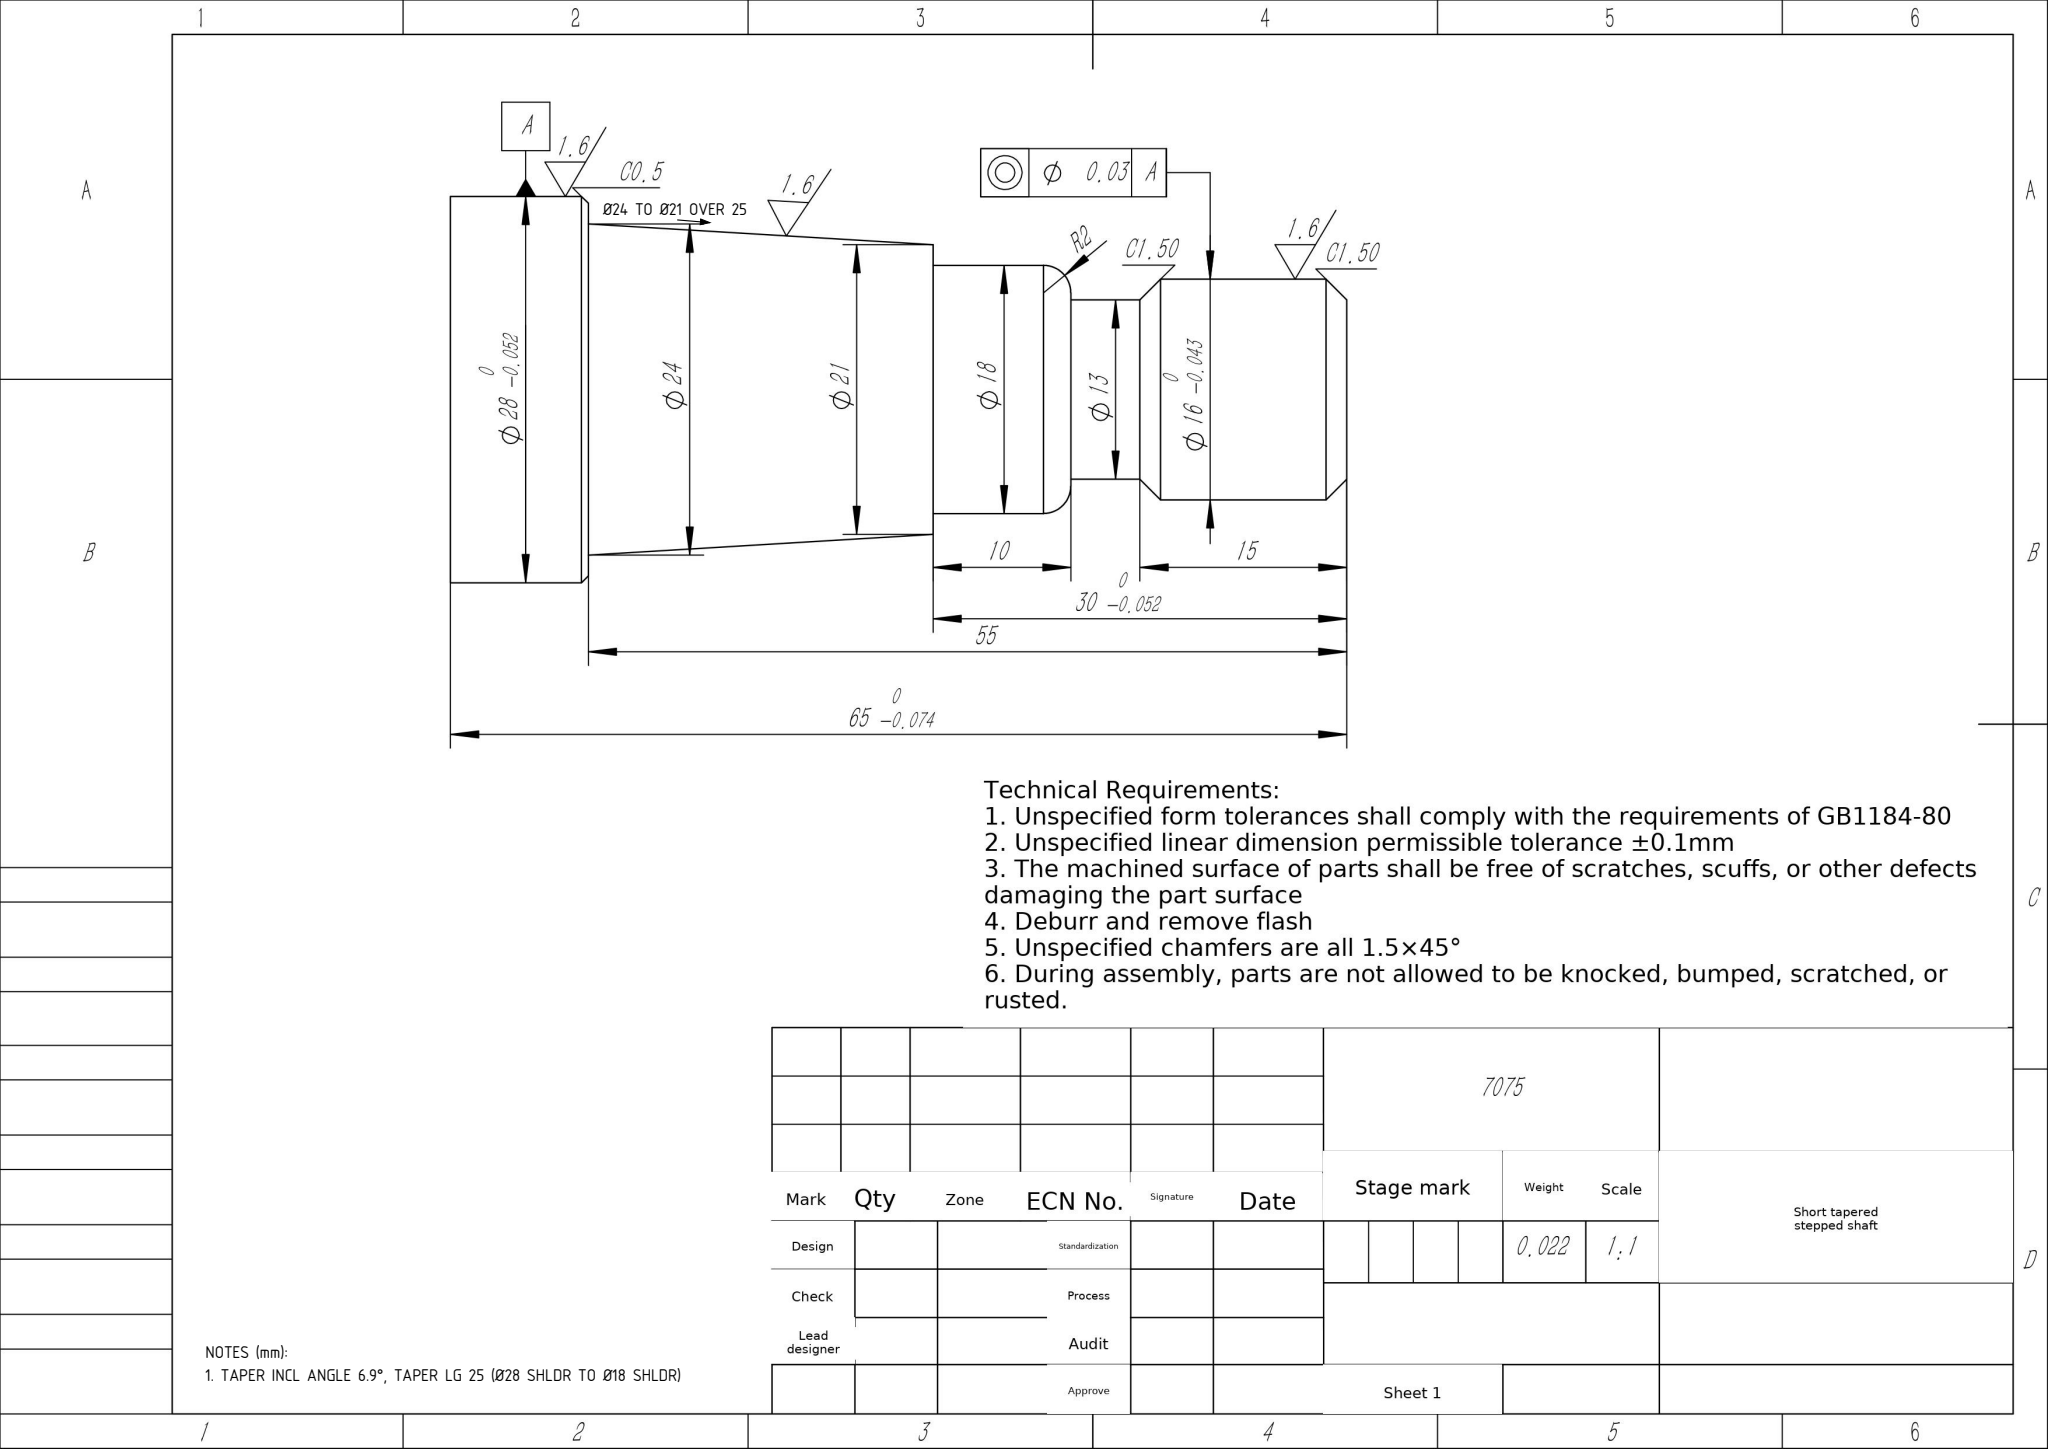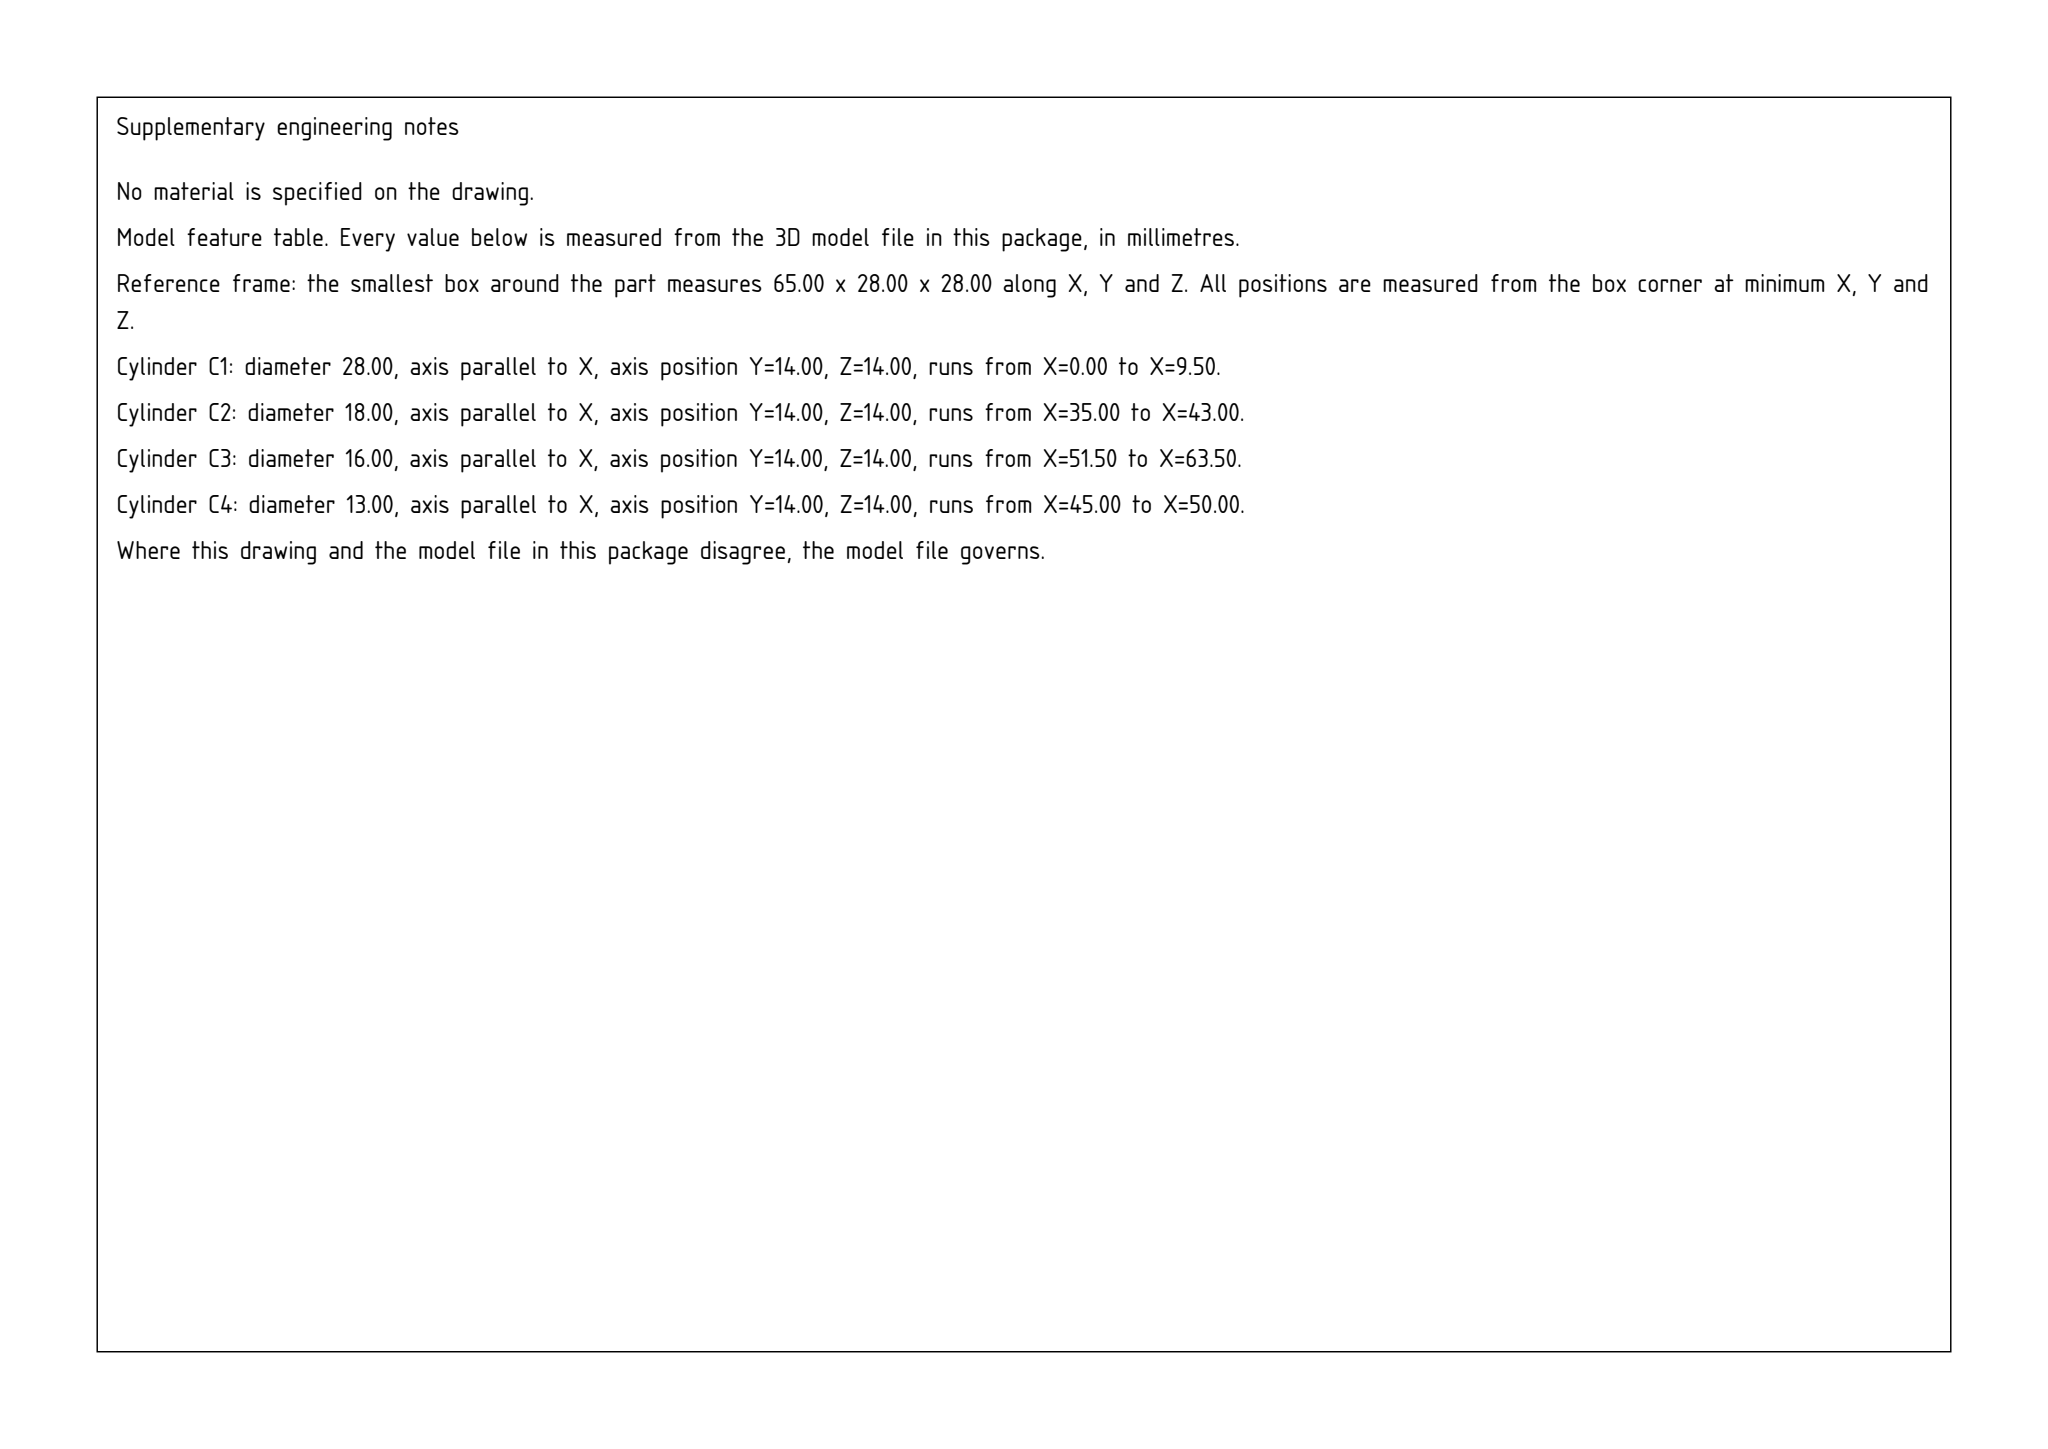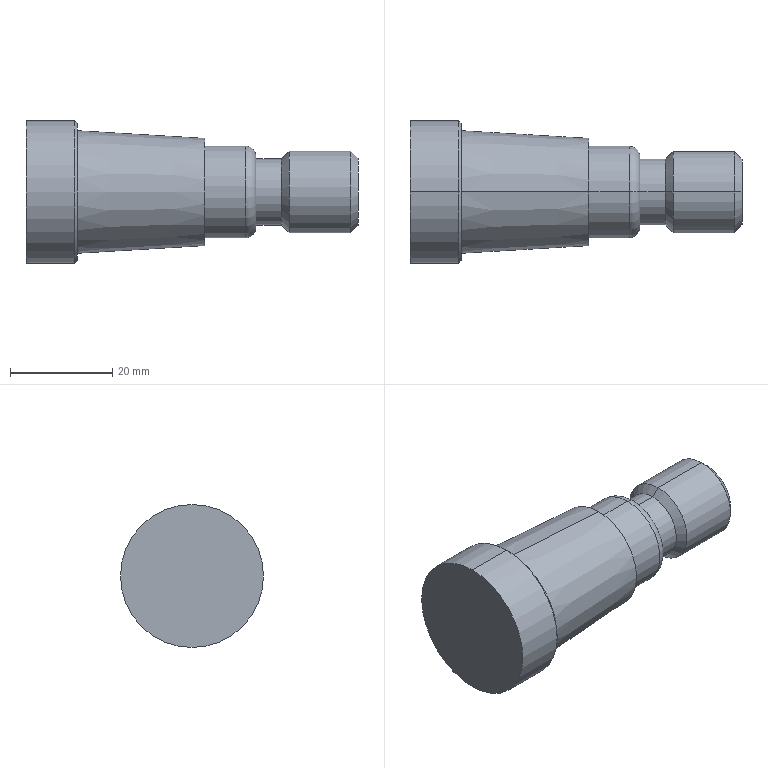Part | SolidWorks | mm | material 7075 | 1 solid | 23 faces | box 65 x 28 x 28 mm | volume 22174 mm3 | cone 8 | cylinder 8 | plane 5 | torus 2 | commonest cylinder face diameters 16 x2 13 x2 18 x2 28 x2
Drawing notes:
TAPER: Ø24 AT Ø28 SHLDR FACE, Ø21 AT 25 FROM THAT FACE | from the solid: Cone ref dia 21, spans planes x=10 to x=35; Ø28 cyl ends x=9.5/face x=10; dia change 3 over 25
TAPER INCL ANGLE 6.9°, TAPER LG 25 (Ø28 SHLDR TO Ø18 SHLDR) | from the solid: cones[included_angle,ref_dia]=[6.9,21]; axis planes x=10 and x=35 -> 25 long
STEP:
#1=CARTESIAN_POINT('',(10.,0.,-13.5));
#2=VERTEX_POINT('',#1);
#3=CARTESIAN_POINT('',(10.,0.,13.5));
#4=VERTEX_POINT('',#3);
#5=CARTESIAN_POINT('',(10.,0.,0.));
#6=DIRECTION('',(1.,0.,0.));
#7=DIRECTION('',(0.,0.,1.));
#8=AXIS2_PLACEMENT_3D('',#5,#6,#7);
#9=CIRCLE('',#8,13.5);
#10=EDGE_CURVE('',#2,#4,#9,.T.);
#11=ORIENTED_EDGE('',*,*,#10,.F.);
#12=CARTESIAN_POINT('',(9.5,0.,-14.));
#13=VERTEX_POINT('',#12);
#14=CARTESIAN_POINT('',(9.5,0.,-14.));
#15=DIRECTION('',(-0.7071,0.,-0.7071));
#16=VECTOR('',#15,1000.);
#17=LINE('',#14,#16);
#18=EDGE_CURVE('',#2,#13,#17,.T.);
#19=ORIENTED_EDGE('',*,*,#18,.T.);
#20=CARTESIAN_POINT('',(9.5,0.,14.));
#21=VERTEX_POINT('',#20);
#22=CARTESIAN_POINT('',(9.5,0.,0.));
#23=DIRECTION('',(-1.,0.,0.));
#24=DIRECTION('',(0.,0.,1.));
#25=AXIS2_PLACEMENT_3D('',#22,#23,#24);
#26=CIRCLE('',#25,14.);
#27=EDGE_CURVE('',#21,#13,#26,.T.);
#28=ORIENTED_EDGE('',*,*,#27,.F.);
#29=CARTESIAN_POINT('',(9.5,0.,14.));
#30=DIRECTION('',(-0.7071,0.,0.7071));
#31=VECTOR('',#30,1000.);
#32=LINE('',#29,#31);
#33=EDGE_CURVE('',#4,#21,#32,.T.);
#34=ORIENTED_EDGE('',*,*,#33,.F.);
#35=EDGE_LOOP('',(#11,#19,#28,#34));
#36=FACE_OUTER_BOUND('',#35,.T.);
#37=CARTESIAN_POINT('',(9.5,0.,0.));
#38=DIRECTION('',(-1.,0.,0.));
#39=DIRECTION('',(0.,0.,1.));
#40=AXIS2_PLACEMENT_3D('',#37,#38,#39);
#41=CONICAL_SURFACE('',#40,14.,0.7854);
#42=ADVANCED_FACE('',(#36),#41,.T.);
#43=CARTESIAN_POINT('',(45.,0.,-7.));
#44=VERTEX_POINT('',#43);
#45=CARTESIAN_POINT('',(45.,0.,7.));
#46=VERTEX_POINT('',#45);
#47=CARTESIAN_POINT('',(45.,0.,0.));
#48=DIRECTION('',(1.,0.,0.));
#49=DIRECTION('',(0.,0.,1.));
#50=AXIS2_PLACEMENT_3D('',#47,#48,#49);
#51=CIRCLE('',#50,7.);
#52=EDGE_CURVE('',#44,#46,#51,.T.);
#53=ORIENTED_EDGE('',*,*,#52,.F.);
#54=CARTESIAN_POINT('',(43.,0.,-9.));
#55=VERTEX_POINT('',#54);
#56=CARTESIAN_POINT('',(43.,0.,-7.));
#57=DIRECTION('',(0.,1.,0.));
#58=DIRECTION('',(0.,-0.,1.));
#59=AXIS2_PLACEMENT_3D('',#56,#57,#58);
#60=CIRCLE('',#59,2.);
#61=EDGE_CURVE('',#44,#55,#60,.T.);
#62=ORIENTED_EDGE('',*,*,#61,.T.);
#63=CARTESIAN_POINT('',(43.,0.,9.));
#64=VERTEX_POINT('',#63);
#65=CARTESIAN_POINT('',(43.,0.,0.));
#66=DIRECTION('',(-1.,0.,0.));
#67=DIRECTION('',(0.,0.,1.));
#68=AXIS2_PLACEMENT_3D('',#65,#66,#67);
#69=CIRCLE('',#68,9.);
#70=EDGE_CURVE('',#64,#55,#69,.T.);
#71=ORIENTED_EDGE('',*,*,#70,.F.);
#72=CARTESIAN_POINT('',(43.,0.,7.));
#73=DIRECTION('',(0.,-1.,0.));
#74=DIRECTION('',(0.,0.,-1.));
#75=AXIS2_PLACEMENT_3D('',#72,#73,#74);
#76=CIRCLE('',#75,2.);
#77=EDGE_CURVE('',#46,#64,#76,.T.);
#78=ORIENTED_EDGE('',*,*,#77,.F.);
#79=EDGE_LOOP('',(#53,#62,#71,#78));
#80=FACE_OUTER_BOUND('',#79,.T.);
#81=CARTESIAN_POINT('',(43.,0.,0.));
#82=DIRECTION('',(-1.,0.,0.));
#83=DIRECTION('',(0.,0.,1.));
#84=AXIS2_PLACEMENT_3D('',#81,#82,#83);
#85=TOROIDAL_SURFACE('',#84,7.,2.);
#86=ADVANCED_FACE('',(#80),#85,.T.);
#87=CARTESIAN_POINT('',(50.,0.,6.5));
#88=VERTEX_POINT('',#87);
#89=CARTESIAN_POINT('',(50.,0.,-6.5));
#90=VERTEX_POINT('',#89);
#91=CARTESIAN_POINT('',(50.,0.,0.));
#92=DIRECTION('',(-1.,0.,0.));
#93=DIRECTION('',(0.,0.,1.));
#94=AXIS2_PLACEMENT_3D('',#91,#92,#93);
#95=CIRCLE('',#94,6.5);
#96=EDGE_CURVE('',#88,#90,#95,.T.);
#97=ORIENTED_EDGE('',*,*,#96,.F.);
#98=CARTESIAN_POINT('',(51.5,0.,8.));
#99=VERTEX_POINT('',#98);
#100=CARTESIAN_POINT('',(50.,0.,6.5));
#101=DIRECTION('',(0.7071,0.,0.7071));
#102=VECTOR('',#101,1000.);
#103=LINE('',#100,#102);
#104=EDGE_CURVE('',#88,#99,#103,.T.);
#105=ORIENTED_EDGE('',*,*,#104,.T.);
#106=CARTESIAN_POINT('',(51.5,0.,-8.));
#107=VERTEX_POINT('',#106);
#108=CARTESIAN_POINT('',(51.5,0.,0.));
#109=DIRECTION('',(1.,0.,0.));
#110=DIRECTION('',(0.,0.,-1.));
#111=AXIS2_PLACEMENT_3D('',#108,#109,#110);
#112=CIRCLE('',#111,8.);
#113=EDGE_CURVE('',#107,#99,#112,.T.);
#114=ORIENTED_EDGE('',*,*,#113,.F.);
#115=CARTESIAN_POINT('',(50.,0.,-6.5));
#116=DIRECTION('',(0.7071,0.,-0.7071));
#117=VECTOR('',#116,1000.);
#118=LINE('',#115,#117);
#119=EDGE_CURVE('',#90,#107,#118,.T.);
#120=ORIENTED_EDGE('',*,*,#119,.F.);
#121=EDGE_LOOP('',(#97,#105,#114,#120));
#122=FACE_OUTER_BOUND('',#121,.T.);
#123=CARTESIAN_POINT('',(50.,0.,0.));
#124=DIRECTION('',(1.,0.,0.));
#125=DIRECTION('',(0.,0.,-1.));
#126=AXIS2_PLACEMENT_3D('',#123,#124,#125);
#127=CONICAL_SURFACE('',#126,6.5,0.7854);
#128=ADVANCED_FACE('',(#122),#127,.T.);
#129=CARTESIAN_POINT('',(65.,0.,-6.5));
#130=VERTEX_POINT('',#129);
#131=CARTESIAN_POINT('',(65.,0.,6.5));
#132=VERTEX_POINT('',#131);
#133=CARTESIAN_POINT('',(65.,0.,0.));
#134=DIRECTION('',(1.,0.,0.));
#135=DIRECTION('',(0.,0.,1.));
#136=AXIS2_PLACEMENT_3D('',#133,#134,#135);
#137=CIRCLE('',#136,6.5);
#138=EDGE_CURVE('',#130,#132,#137,.T.);
#139=ORIENTED_EDGE('',*,*,#138,.F.);
#140=CARTESIAN_POINT('',(63.5,0.,-8.));
#141=VERTEX_POINT('',#140);
#142=CARTESIAN_POINT('',(63.5,0.,-8.));
#143=DIRECTION('',(-0.7071,0.,-0.7071));
#144=VECTOR('',#143,1000.);
#145=LINE('',#142,#144);
#146=EDGE_CURVE('',#130,#141,#145,.T.);
#147=ORIENTED_EDGE('',*,*,#146,.T.);
#148=CARTESIAN_POINT('',(63.5,0.,8.));
#149=VERTEX_POINT('',#148);
#150=CARTESIAN_POINT('',(63.5,0.,0.));
#151=DIRECTION('',(-1.,0.,0.));
#152=DIRECTION('',(0.,0.,1.));
#153=AXIS2_PLACEMENT_3D('',#150,#151,#152);
#154=CIRCLE('',#153,8.);
#155=EDGE_CURVE('',#149,#141,#154,.T.);
#156=ORIENTED_EDGE('',*,*,#155,.F.);
#157=CARTESIAN_POINT('',(63.5,0.,8.));
#158=DIRECTION('',(-0.7071,0.,0.7071));
#159=VECTOR('',#158,1000.);
#160=LINE('',#157,#159);
#161=EDGE_CURVE('',#132,#149,#160,.T.);
#162=ORIENTED_EDGE('',*,*,#161,.F.);
#163=EDGE_LOOP('',(#139,#147,#156,#162));
#164=FACE_OUTER_BOUND('',#163,.T.);
#165=CARTESIAN_POINT('',(63.5,0.,0.));
#166=DIRECTION('',(-1.,0.,0.));
#167=DIRECTION('',(0.,0.,1.));
#168=AXIS2_PLACEMENT_3D('',#165,#166,#167);
#169=CONICAL_SURFACE('',#168,8.,0.7854);
#170=ADVANCED_FACE('',(#164),#169,.T.);
#171=ORIENTED_EDGE('',*,*,#155,.T.);
#172=CARTESIAN_POINT('',(0.,0.,-8.));
#173=DIRECTION('',(-1.,0.,0.));
#174=VECTOR('',#173,1000.);
#175=LINE('',#172,#174);
#176=EDGE_CURVE('',#141,#107,#175,.T.);
#177=ORIENTED_EDGE('',*,*,#176,.T.);
#178=ORIENTED_EDGE('',*,*,#113,.T.);
#179=CARTESIAN_POINT('',(0.,0.,8.));
#180=DIRECTION('',(-1.,0.,0.));
#181=VECTOR('',#180,1000.);
#182=LINE('',#179,#181);
#183=EDGE_CURVE('',#149,#99,#182,.T.);
#184=ORIENTED_EDGE('',*,*,#183,.F.);
#185=EDGE_LOOP('',(#171,#177,#178,#184));
#186=FACE_OUTER_BOUND('',#185,.T.);
#187=CARTESIAN_POINT('',(0.,0.,0.));
#188=DIRECTION('',(-1.,0.,0.));
#189=DIRECTION('',(0.,0.,1.));
#190=AXIS2_PLACEMENT_3D('',#187,#188,#189);
#191=CYLINDRICAL_SURFACE('',#190,8.);
#192=ADVANCED_FACE('',(#186),#191,.T.);
#193=ORIENTED_EDGE('',*,*,#96,.T.);
#194=CARTESIAN_POINT('',(45.,0.,-6.5));
#195=VERTEX_POINT('',#194);
#196=CARTESIAN_POINT('',(0.,0.,-6.5));
#197=DIRECTION('',(-1.,0.,0.));
#198=VECTOR('',#197,1000.);
#199=LINE('',#196,#198);
#200=EDGE_CURVE('',#90,#195,#199,.T.);
#201=ORIENTED_EDGE('',*,*,#200,.T.);
#202=CARTESIAN_POINT('',(45.,0.,6.5));
#203=VERTEX_POINT('',#202);
#204=CARTESIAN_POINT('',(45.,0.,0.));
#205=DIRECTION('',(-1.,0.,0.));
#206=DIRECTION('',(0.,0.,1.));
#207=AXIS2_PLACEMENT_3D('',#204,#205,#206);
#208=CIRCLE('',#207,6.5);
#209=EDGE_CURVE('',#203,#195,#208,.T.);
#210=ORIENTED_EDGE('',*,*,#209,.F.);
#211=CARTESIAN_POINT('',(0.,0.,6.5));
#212=DIRECTION('',(-1.,0.,0.));
#213=VECTOR('',#212,1000.);
#214=LINE('',#211,#213);
#215=EDGE_CURVE('',#88,#203,#214,.T.);
#216=ORIENTED_EDGE('',*,*,#215,.F.);
#217=EDGE_LOOP('',(#193,#201,#210,#216));
#218=FACE_OUTER_BOUND('',#217,.T.);
#219=CARTESIAN_POINT('',(0.,0.,0.));
#220=DIRECTION('',(-1.,0.,0.));
#221=DIRECTION('',(0.,0.,1.));
#222=AXIS2_PLACEMENT_3D('',#219,#220,#221);
#223=CYLINDRICAL_SURFACE('',#222,6.5);
#224=ADVANCED_FACE('',(#218),#223,.T.);
#225=ORIENTED_EDGE('',*,*,#70,.T.);
#226=CARTESIAN_POINT('',(35.,0.,-9.));
#227=VERTEX_POINT('',#226);
#228=CARTESIAN_POINT('',(0.,0.,-9.));
#229=DIRECTION('',(-1.,0.,0.));
#230=VECTOR('',#229,1000.);
#231=LINE('',#228,#230);
#232=EDGE_CURVE('',#55,#227,#231,.T.);
#233=ORIENTED_EDGE('',*,*,#232,.T.);
#234=CARTESIAN_POINT('',(35.,0.,9.));
#235=VERTEX_POINT('',#234);
#236=CARTESIAN_POINT('',(35.,0.,0.));
#237=DIRECTION('',(-1.,0.,0.));
#238=DIRECTION('',(0.,0.,1.));
#239=AXIS2_PLACEMENT_3D('',#236,#237,#238);
#240=CIRCLE('',#239,9.);
#241=EDGE_CURVE('',#235,#227,#240,.T.);
#242=ORIENTED_EDGE('',*,*,#241,.F.);
#243=CARTESIAN_POINT('',(0.,0.,9.));
#244=DIRECTION('',(-1.,0.,0.));
#245=VECTOR('',#244,1000.);
#246=LINE('',#243,#245);
#247=EDGE_CURVE('',#64,#235,#246,.T.);
#248=ORIENTED_EDGE('',*,*,#247,.F.);
#249=EDGE_LOOP('',(#225,#233,#242,#248));
#250=FACE_OUTER_BOUND('',#249,.T.);
#251=CARTESIAN_POINT('',(0.,0.,0.));
#252=DIRECTION('',(-1.,0.,0.));
#253=DIRECTION('',(0.,0.,1.));
#254=AXIS2_PLACEMENT_3D('',#251,#252,#253);
#255=CYLINDRICAL_SURFACE('',#254,9.);
#256=ADVANCED_FACE('',(#250),#255,.T.);
#257=CARTESIAN_POINT('',(35.,0.,10.5));
#258=VERTEX_POINT('',#257);
#259=CARTESIAN_POINT('',(35.,0.,-10.5));
#260=VERTEX_POINT('',#259);
#261=CARTESIAN_POINT('',(35.,0.,0.));
#262=DIRECTION('',(-1.,0.,0.));
#263=DIRECTION('',(0.,0.,1.));
#264=AXIS2_PLACEMENT_3D('',#261,#262,#263);
#265=CIRCLE('',#264,10.5);
#266=EDGE_CURVE('',#258,#260,#265,.T.);
#267=ORIENTED_EDGE('',*,*,#266,.T.);
#268=CARTESIAN_POINT('',(10.,0.,-12.));
#269=VERTEX_POINT('',#268);
#270=CARTESIAN_POINT('',(35.,0.,-10.5));
#271=DIRECTION('',(-0.9982,0.,-0.05989));
#272=VECTOR('',#271,1000.);
#273=LINE('',#270,#272);
#274=EDGE_CURVE('',#260,#269,#273,.T.);
#275=ORIENTED_EDGE('',*,*,#274,.T.);
#276=CARTESIAN_POINT('',(10.,0.,12.));
#277=VERTEX_POINT('',#276);
#278=CARTESIAN_POINT('',(10.,0.,0.));
#279=DIRECTION('',(-1.,0.,0.));
#280=DIRECTION('',(0.,0.,1.));
#281=AXIS2_PLACEMENT_3D('',#278,#279,#280);
#282=CIRCLE('',#281,12.);
#283=EDGE_CURVE('',#277,#269,#282,.T.);
#284=ORIENTED_EDGE('',*,*,#283,.F.);
#285=CARTESIAN_POINT('',(35.,0.,10.5));
#286=DIRECTION('',(-0.9982,0.,0.05989));
#287=VECTOR('',#286,1000.);
#288=LINE('',#285,#287);
#289=EDGE_CURVE('',#258,#277,#288,.T.);
#290=ORIENTED_EDGE('',*,*,#289,.F.);
#291=EDGE_LOOP('',(#267,#275,#284,#290));
#292=FACE_OUTER_BOUND('',#291,.T.);
#293=CARTESIAN_POINT('',(35.,0.,0.));
#294=DIRECTION('',(-1.,0.,0.));
#295=DIRECTION('',(0.,0.,1.));
#296=AXIS2_PLACEMENT_3D('',#293,#294,#295);
#297=CONICAL_SURFACE('',#296,10.5,0.05993);
#298=ADVANCED_FACE('',(#292),#297,.T.);
#299=ORIENTED_EDGE('',*,*,#27,.T.);
#300=CARTESIAN_POINT('',(0.,0.,-14.));
#301=VERTEX_POINT('',#300);
#302=CARTESIAN_POINT('',(0.,0.,-14.));
#303=DIRECTION('',(-1.,0.,0.));
#304=VECTOR('',#303,1000.);
#305=LINE('',#302,#304);
#306=EDGE_CURVE('',#13,#301,#305,.T.);
#307=ORIENTED_EDGE('',*,*,#306,.T.);
#308=CARTESIAN_POINT('',(0.,0.,14.));
#309=VERTEX_POINT('',#308);
#310=CARTESIAN_POINT('',(0.,0.,0.));
#311=DIRECTION('',(-1.,0.,0.));
#312=DIRECTION('',(0.,0.,1.));
#313=AXIS2_PLACEMENT_3D('',#310,#311,#312);
#314=CIRCLE('',#313,14.);
#315=EDGE_CURVE('',#309,#301,#314,.T.);
#316=ORIENTED_EDGE('',*,*,#315,.F.);
#317=CARTESIAN_POINT('',(0.,0.,14.));
#318=DIRECTION('',(-1.,0.,0.));
#319=VECTOR('',#318,1000.);
#320=LINE('',#317,#319);
#321=EDGE_CURVE('',#21,#309,#320,.T.);
#322=ORIENTED_EDGE('',*,*,#321,.F.);
#323=EDGE_LOOP('',(#299,#307,#316,#322));
#324=FACE_OUTER_BOUND('',#323,.T.);
#325=CARTESIAN_POINT('',(0.,0.,0.));
#326=DIRECTION('',(-1.,0.,0.));
#327=DIRECTION('',(0.,0.,1.));
#328=AXIS2_PLACEMENT_3D('',#325,#326,#327);
#329=CYLINDRICAL_SURFACE('',#328,14.);
#330=ADVANCED_FACE('',(#324),#329,.T.);
#331=ORIENTED_EDGE('',*,*,#315,.T.);
#332=CARTESIAN_POINT('',(0.,0.,0.));
#333=DIRECTION('',(-1.,0.,0.));
#334=DIRECTION('',(0.,0.,1.));
#335=AXIS2_PLACEMENT_3D('',#332,#333,#334);
#336=CIRCLE('',#335,14.);
#337=EDGE_CURVE('',#301,#309,#336,.T.);
#338=ORIENTED_EDGE('',*,*,#337,.T.);
#339=EDGE_LOOP('',(#331,#338));
#340=FACE_OUTER_BOUND('',#339,.T.);
#341=CARTESIAN_POINT('',(0.,0.,0.));
#342=DIRECTION('',(1.,0.,0.));
#343=DIRECTION('',(0.,0.,-1.));
#344=AXIS2_PLACEMENT_3D('',#341,#342,#343);
#345=PLANE('',#344);
#346=ADVANCED_FACE('',(#340),#345,.F.);
#347=ORIENTED_EDGE('',*,*,#306,.F.);
#348=CARTESIAN_POINT('',(9.5,0.,0.));
#349=DIRECTION('',(-1.,0.,0.));
#350=DIRECTION('',(0.,0.,1.));
#351=AXIS2_PLACEMENT_3D('',#348,#349,#350);
#352=CIRCLE('',#351,14.);
#353=EDGE_CURVE('',#13,#21,#352,.T.);
#354=ORIENTED_EDGE('',*,*,#353,.T.);
#355=ORIENTED_EDGE('',*,*,#321,.T.);
#356=ORIENTED_EDGE('',*,*,#337,.F.);
#357=EDGE_LOOP('',(#347,#354,#355,#356));
#358=FACE_OUTER_BOUND('',#357,.T.);
#359=CARTESIAN_POINT('',(0.,0.,0.));
#360=DIRECTION('',(-1.,0.,0.));
#361=DIRECTION('',(0.,0.,1.));
#362=AXIS2_PLACEMENT_3D('',#359,#360,#361);
#363=CYLINDRICAL_SURFACE('',#362,14.);
#364=ADVANCED_FACE('',(#358),#363,.T.);
#365=CARTESIAN_POINT('',(10.,0.,0.));
#366=DIRECTION('',(1.,0.,0.));
#367=DIRECTION('',(0.,0.,1.));
#368=AXIS2_PLACEMENT_3D('',#365,#366,#367);
#369=CIRCLE('',#368,13.5);
#370=EDGE_CURVE('',#4,#2,#369,.T.);
#371=ORIENTED_EDGE('',*,*,#370,.T.);
#372=ORIENTED_EDGE('',*,*,#10,.T.);
#373=EDGE_LOOP('',(#371,#372));
#374=FACE_OUTER_BOUND('',#373,.T.);
#375=ORIENTED_EDGE('',*,*,#283,.T.);
#376=CARTESIAN_POINT('',(10.,0.,0.));
#377=DIRECTION('',(-1.,0.,0.));
#378=DIRECTION('',(0.,0.,1.));
#379=AXIS2_PLACEMENT_3D('',#376,#377,#378);
#380=CIRCLE('',#379,12.);
#381=EDGE_CURVE('',#269,#277,#380,.T.);
#382=ORIENTED_EDGE('',*,*,#381,.T.);
#383=EDGE_LOOP('',(#375,#382));
#384=FACE_BOUND('',#383,.T.);
#385=CARTESIAN_POINT('',(10.,14.,0.));
#386=DIRECTION('',(-1.,0.,0.));
#387=DIRECTION('',(0.,0.,1.));
#388=AXIS2_PLACEMENT_3D('',#385,#386,#387);
#389=PLANE('',#388);
#390=ADVANCED_FACE('',(#374,#384),#389,.F.);
#391=ORIENTED_EDGE('',*,*,#274,.F.);
#392=CARTESIAN_POINT('',(35.,0.,0.));
#393=DIRECTION('',(-1.,0.,0.));
#394=DIRECTION('',(0.,0.,1.));
#395=AXIS2_PLACEMENT_3D('',#392,#393,#394);
#396=CIRCLE('',#395,10.5);
#397=EDGE_CURVE('',#260,#258,#396,.T.);
#398=ORIENTED_EDGE('',*,*,#397,.T.);
#399=ORIENTED_EDGE('',*,*,#289,.T.);
#400=ORIENTED_EDGE('',*,*,#381,.F.);
#401=EDGE_LOOP('',(#391,#398,#399,#400));
#402=FACE_OUTER_BOUND('',#401,.T.);
#403=CARTESIAN_POINT('',(35.,0.,0.));
#404=DIRECTION('',(-1.,0.,0.));
#405=DIRECTION('',(0.,0.,1.));
#406=AXIS2_PLACEMENT_3D('',#403,#404,#405);
#407=CONICAL_SURFACE('',#406,10.5,0.05993);
#408=ADVANCED_FACE('',(#402),#407,.T.);
#409=ORIENTED_EDGE('',*,*,#266,.F.);
#410=ORIENTED_EDGE('',*,*,#397,.F.);
#411=EDGE_LOOP('',(#409,#410));
#412=FACE_OUTER_BOUND('',#411,.T.);
#413=ORIENTED_EDGE('',*,*,#241,.T.);
#414=CARTESIAN_POINT('',(35.,0.,0.));
#415=DIRECTION('',(-1.,0.,0.));
#416=DIRECTION('',(0.,0.,1.));
#417=AXIS2_PLACEMENT_3D('',#414,#415,#416);
#418=CIRCLE('',#417,9.);
#419=EDGE_CURVE('',#227,#235,#418,.T.);
#420=ORIENTED_EDGE('',*,*,#419,.T.);
#421=EDGE_LOOP('',(#413,#420));
#422=FACE_BOUND('',#421,.T.);
#423=CARTESIAN_POINT('',(35.,10.5,0.));
#424=DIRECTION('',(-1.,0.,0.));
#425=DIRECTION('',(0.,0.,1.));
#426=AXIS2_PLACEMENT_3D('',#423,#424,#425);
#427=PLANE('',#426);
#428=ADVANCED_FACE('',(#412,#422),#427,.F.);
#429=ORIENTED_EDGE('',*,*,#232,.F.);
#430=CARTESIAN_POINT('',(43.,0.,0.));
#431=DIRECTION('',(-1.,0.,0.));
#432=DIRECTION('',(0.,0.,1.));
#433=AXIS2_PLACEMENT_3D('',#430,#431,#432);
#434=CIRCLE('',#433,9.);
#435=EDGE_CURVE('',#55,#64,#434,.T.);
#436=ORIENTED_EDGE('',*,*,#435,.T.);
#437=ORIENTED_EDGE('',*,*,#247,.T.);
#438=ORIENTED_EDGE('',*,*,#419,.F.);
#439=EDGE_LOOP('',(#429,#436,#437,#438));
#440=FACE_OUTER_BOUND('',#439,.T.);
#441=CARTESIAN_POINT('',(0.,0.,0.));
#442=DIRECTION('',(-1.,0.,0.));
#443=DIRECTION('',(0.,0.,1.));
#444=AXIS2_PLACEMENT_3D('',#441,#442,#443);
#445=CYLINDRICAL_SURFACE('',#444,9.);
#446=ADVANCED_FACE('',(#440),#445,.T.);
#447=CARTESIAN_POINT('',(45.,0.,0.));
#448=DIRECTION('',(1.,0.,0.));
#449=DIRECTION('',(0.,0.,1.));
#450=AXIS2_PLACEMENT_3D('',#447,#448,#449);
#451=CIRCLE('',#450,7.);
#452=EDGE_CURVE('',#46,#44,#451,.T.);
#453=ORIENTED_EDGE('',*,*,#452,.T.);
#454=ORIENTED_EDGE('',*,*,#52,.T.);
#455=EDGE_LOOP('',(#453,#454));
#456=FACE_OUTER_BOUND('',#455,.T.);
#457=ORIENTED_EDGE('',*,*,#209,.T.);
#458=CARTESIAN_POINT('',(45.,0.,0.));
#459=DIRECTION('',(-1.,0.,0.));
#460=DIRECTION('',(0.,0.,1.));
#461=AXIS2_PLACEMENT_3D('',#458,#459,#460);
#462=CIRCLE('',#461,6.5);
#463=EDGE_CURVE('',#195,#203,#462,.T.);
#464=ORIENTED_EDGE('',*,*,#463,.T.);
#465=EDGE_LOOP('',(#457,#464));
#466=FACE_BOUND('',#465,.T.);
#467=CARTESIAN_POINT('',(45.,9.,0.));
#468=DIRECTION('',(-1.,0.,0.));
#469=DIRECTION('',(0.,0.,1.));
#470=AXIS2_PLACEMENT_3D('',#467,#468,#469);
#471=PLANE('',#470);
#472=ADVANCED_FACE('',(#456,#466),#471,.F.);
#473=ORIENTED_EDGE('',*,*,#200,.F.);
#474=CARTESIAN_POINT('',(50.,0.,0.));
#475=DIRECTION('',(-1.,0.,0.));
#476=DIRECTION('',(0.,0.,1.));
#477=AXIS2_PLACEMENT_3D('',#474,#475,#476);
#478=CIRCLE('',#477,6.5);
#479=EDGE_CURVE('',#90,#88,#478,.T.);
#480=ORIENTED_EDGE('',*,*,#479,.T.);
#481=ORIENTED_EDGE('',*,*,#215,.T.);
#482=ORIENTED_EDGE('',*,*,#463,.F.);
#483=EDGE_LOOP('',(#473,#480,#481,#482));
#484=FACE_OUTER_BOUND('',#483,.T.);
#485=CARTESIAN_POINT('',(0.,0.,0.));
#486=DIRECTION('',(-1.,0.,0.));
#487=DIRECTION('',(0.,0.,1.));
#488=AXIS2_PLACEMENT_3D('',#485,#486,#487);
#489=CYLINDRICAL_SURFACE('',#488,6.5);
#490=ADVANCED_FACE('',(#484),#489,.T.);
#491=ORIENTED_EDGE('',*,*,#176,.F.);
#492=CARTESIAN_POINT('',(63.5,0.,0.));
#493=DIRECTION('',(-1.,0.,0.));
#494=DIRECTION('',(0.,0.,1.));
#495=AXIS2_PLACEMENT_3D('',#492,#493,#494);
#496=CIRCLE('',#495,8.);
#497=EDGE_CURVE('',#141,#149,#496,.T.);
#498=ORIENTED_EDGE('',*,*,#497,.T.);
#499=ORIENTED_EDGE('',*,*,#183,.T.);
#500=CARTESIAN_POINT('',(51.5,0.,0.));
#501=DIRECTION('',(1.,0.,0.));
#502=DIRECTION('',(0.,0.,-1.));
#503=AXIS2_PLACEMENT_3D('',#500,#501,#502);
#504=CIRCLE('',#503,8.);
#505=EDGE_CURVE('',#99,#107,#504,.T.);
#506=ORIENTED_EDGE('',*,*,#505,.T.);
#507=EDGE_LOOP('',(#491,#498,#499,#506));
#508=FACE_OUTER_BOUND('',#507,.T.);
#509=CARTESIAN_POINT('',(0.,0.,0.));
#510=DIRECTION('',(-1.,0.,0.));
#511=DIRECTION('',(0.,0.,1.));
#512=AXIS2_PLACEMENT_3D('',#509,#510,#511);
#513=CYLINDRICAL_SURFACE('',#512,8.);
#514=ADVANCED_FACE('',(#508),#513,.T.);
#515=CARTESIAN_POINT('',(65.,0.,0.));
#516=DIRECTION('',(1.,0.,0.));
#517=DIRECTION('',(0.,0.,1.));
#518=AXIS2_PLACEMENT_3D('',#515,#516,#517);
#519=CIRCLE('',#518,6.5);
#520=EDGE_CURVE('',#132,#130,#519,.T.);
#521=ORIENTED_EDGE('',*,*,#520,.T.);
#522=ORIENTED_EDGE('',*,*,#138,.T.);
#523=EDGE_LOOP('',(#521,#522));
#524=FACE_OUTER_BOUND('',#523,.T.);
#525=CARTESIAN_POINT('',(65.,8.,0.));
#526=DIRECTION('',(-1.,0.,0.));
#527=DIRECTION('',(0.,0.,1.));
#528=AXIS2_PLACEMENT_3D('',#525,#526,#527);
#529=PLANE('',#528);
#530=ADVANCED_FACE('',(#524),#529,.F.);
#531=ORIENTED_EDGE('',*,*,#146,.F.);
#532=ORIENTED_EDGE('',*,*,#520,.F.);
#533=ORIENTED_EDGE('',*,*,#161,.T.);
#534=ORIENTED_EDGE('',*,*,#497,.F.);
#535=EDGE_LOOP('',(#531,#532,#533,#534));
#536=FACE_OUTER_BOUND('',#535,.T.);
#537=CARTESIAN_POINT('',(63.5,0.,0.));
#538=DIRECTION('',(-1.,0.,0.));
#539=DIRECTION('',(0.,0.,1.));
#540=AXIS2_PLACEMENT_3D('',#537,#538,#539);
#541=CONICAL_SURFACE('',#540,8.,0.7854);
#542=ADVANCED_FACE('',(#536),#541,.T.);
#543=ORIENTED_EDGE('',*,*,#104,.F.);
#544=ORIENTED_EDGE('',*,*,#479,.F.);
#545=ORIENTED_EDGE('',*,*,#119,.T.);
#546=ORIENTED_EDGE('',*,*,#505,.F.);
#547=EDGE_LOOP('',(#543,#544,#545,#546));
#548=FACE_OUTER_BOUND('',#547,.T.);
#549=CARTESIAN_POINT('',(50.,0.,0.));
#550=DIRECTION('',(1.,0.,0.));
#551=DIRECTION('',(0.,0.,-1.));
#552=AXIS2_PLACEMENT_3D('',#549,#550,#551);
#553=CONICAL_SURFACE('',#552,6.5,0.7854);
#554=ADVANCED_FACE('',(#548),#553,.T.);
#555=ORIENTED_EDGE('',*,*,#61,.F.);
#556=ORIENTED_EDGE('',*,*,#452,.F.);
#557=ORIENTED_EDGE('',*,*,#77,.T.);
#558=ORIENTED_EDGE('',*,*,#435,.F.);
#559=EDGE_LOOP('',(#555,#556,#557,#558));
#560=FACE_OUTER_BOUND('',#559,.T.);
#561=CARTESIAN_POINT('',(43.,0.,0.));
#562=DIRECTION('',(-1.,0.,0.));
#563=DIRECTION('',(0.,0.,1.));
#564=AXIS2_PLACEMENT_3D('',#561,#562,#563);
#565=TOROIDAL_SURFACE('',#564,7.,2.);
#566=ADVANCED_FACE('',(#560),#565,.T.);
#567=ORIENTED_EDGE('',*,*,#18,.F.);
#568=ORIENTED_EDGE('',*,*,#370,.F.);
#569=ORIENTED_EDGE('',*,*,#33,.T.);
#570=ORIENTED_EDGE('',*,*,#353,.F.);
#571=EDGE_LOOP('',(#567,#568,#569,#570));
#572=FACE_OUTER_BOUND('',#571,.T.);
#573=CARTESIAN_POINT('',(9.5,0.,0.));
#574=DIRECTION('',(-1.,0.,0.));
#575=DIRECTION('',(0.,0.,1.));
#576=AXIS2_PLACEMENT_3D('',#573,#574,#575);
#577=CONICAL_SURFACE('',#576,14.,0.7854);
#578=ADVANCED_FACE('',(#572),#577,.T.);
#579=CLOSED_SHELL('',(#42,#86,#128,#170,#192,#224,#256,#298,#330,#346,#364,#390,#408,#428,#446,#472,#490,#514,#530,#542,#554,#566,#578));
#580=MANIFOLD_SOLID_BREP('',#579);
#581=CARTESIAN_POINT('',(0.,0.,0.));
#582=DIRECTION('',(0.,0.,1.));
#583=DIRECTION('',(1.,0.,0.));
#584=AXIS2_PLACEMENT_3D('',#581,#582,#583);
#585=(LENGTH_UNIT()NAMED_UNIT(*)SI_UNIT(.MILLI.,.METRE.));
#586=UNCERTAINTY_MEASURE_WITH_UNIT(LENGTH_MEASURE(0.00001),#585,'','');
#587=(NAMED_UNIT(*)PLANE_ANGLE_UNIT()SI_UNIT($,.RADIAN.));
#588=(NAMED_UNIT(*)SI_UNIT($,.STERADIAN.)SOLID_ANGLE_UNIT());
#589=(GEOMETRIC_REPRESENTATION_CONTEXT(3)GLOBAL_UNCERTAINTY_ASSIGNED_CONTEXT((#586))GLOBAL_UNIT_ASSIGNED_CONTEXT((#585,#587,#588))REPRESENTATION_CONTEXT('',''));
#590=ADVANCED_BREP_SHAPE_REPRESENTATION('',(#580,#584),#589);